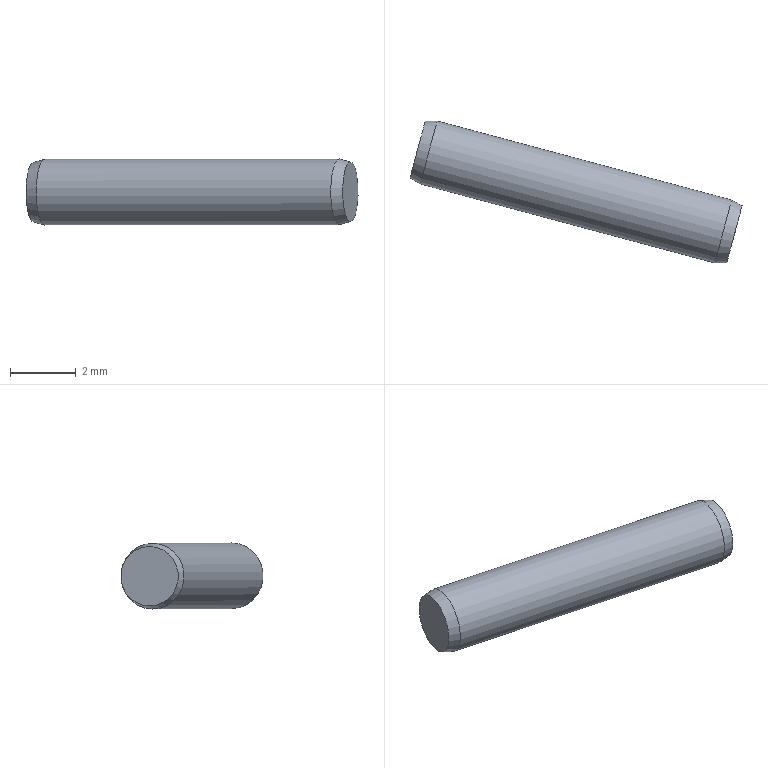Component | NX | GB-T119_1-2000_2X10 | 1 solid | 5 faces | box 10.13 x 4.34 x 2.01 mm | volume 31 mm3 | plane 2 | cone 2 | cylinder 1 | commonest cylinder face diameters 2 x1
STEP:
#1=CARTESIAN_POINT('',(0.,0.,0.));
#2=DIRECTION('',(0.,0.,1.));
#3=DIRECTION('',(1.,0.,0.));
#4=AXIS2_PLACEMENT_3D('',#1,#2,#3);
#5=CARTESIAN_POINT('',(19.96,-124.109,157.371));
#6=VERTEX_POINT('',#5);
#7=CARTESIAN_POINT('',(19.961,-124.109,156.465));
#8=DIRECTION('',(-0.9659,0.2589,-0.001382));
#9=DIRECTION('',(-0.001431,0.,1.));
#10=AXIS2_PLACEMENT_3D('',#7,#8,#9);
#11=CIRCLE('',#10,0.9062);
#12=CARTESIAN_POINT('',(19.961,-124.109,156.465));
#13=DIRECTION('',(-0.9659,0.2589,-0.001382));
#14=DIRECTION('',(-0.001431,-0.,1.));
#15=AXIS2_PLACEMENT_3D('',#12,#13,#14);
#16=PLANE('',#15);
#17=CARTESIAN_POINT('',(0.,0.));
#18=DIRECTION('',(1.,0.));
#19=AXIS2_PLACEMENT_2D('',#17,#18);
#20=CIRCLE('',#19,0.9062);
#21=(GEOMETRIC_REPRESENTATION_CONTEXT(2)PARAMETRIC_REPRESENTATION_CONTEXT()REPRESENTATION_CONTEXT('',''));
#22=DEFINITIONAL_REPRESENTATION('',(#20),#21);
#23=PCURVE('',#16,#22);
#24=CARTESIAN_POINT('',(19.961,-124.109,156.465));
#25=DIRECTION('',(0.9659,-0.2589,0.001382));
#26=DIRECTION('',(0.001431,0.,-1.));
#27=AXIS2_PLACEMENT_3D('',#24,#25,#26);
#28=CONICAL_SURFACE('',#27,0.9062,0.2618);
#29=CARTESIAN_POINT('',(9.425,-0.));
#30=DIRECTION('',(-1.,0.));
#31=VECTOR('',#30,1.);
#32=LINE('',#29,#31);
#33=(GEOMETRIC_REPRESENTATION_CONTEXT(2)PARAMETRIC_REPRESENTATION_CONTEXT()REPRESENTATION_CONTEXT('',''));
#34=DEFINITIONAL_REPRESENTATION('',(#32),#33);
#35=PCURVE('',#28,#34);
#36=SURFACE_CURVE('',#11,(#23,#35),.PCURVE_S1.);
#37=EDGE_CURVE('',#6,#6,#36,.T.);
#38=ORIENTED_EDGE('',*,*,#37,.T.);
#39=EDGE_LOOP('',(#38));
#40=FACE_BOUND('',#39,.T.);
#41=ADVANCED_FACE('',(#40),#16,.T.);
#42=CARTESIAN_POINT('',(20.298,-124.199,157.465));
#43=VERTEX_POINT('',#42);
#44=CARTESIAN_POINT('',(20.299,-124.199,156.465));
#45=DIRECTION('',(-0.9659,0.2589,-0.001382));
#46=DIRECTION('',(-0.001431,-0.,1.));
#47=AXIS2_PLACEMENT_3D('',#44,#45,#46);
#48=CIRCLE('',#47,1.);
#49=CARTESIAN_POINT('',(9.425,0.35));
#50=DIRECTION('',(-1.,0.));
#51=VECTOR('',#50,1.);
#52=LINE('',#49,#51);
#53=(GEOMETRIC_REPRESENTATION_CONTEXT(2)PARAMETRIC_REPRESENTATION_CONTEXT()REPRESENTATION_CONTEXT('',''));
#54=DEFINITIONAL_REPRESENTATION('',(#52),#53);
#55=PCURVE('',#28,#54);
#56=CARTESIAN_POINT('',(29.62,-126.698,156.479));
#57=DIRECTION('',(-0.9659,0.2589,-0.001382));
#58=DIRECTION('',(-0.001431,-0.,1.));
#59=AXIS2_PLACEMENT_3D('',#56,#57,#58);
#60=CYLINDRICAL_SURFACE('',#59,1.);
#61=CARTESIAN_POINT('',(0.,9.65));
#62=DIRECTION('',(1.,0.));
#63=VECTOR('',#62,1.);
#64=LINE('',#61,#63);
#65=(GEOMETRIC_REPRESENTATION_CONTEXT(2)PARAMETRIC_REPRESENTATION_CONTEXT()REPRESENTATION_CONTEXT('',''));
#66=DEFINITIONAL_REPRESENTATION('',(#64),#65);
#67=PCURVE('',#60,#66);
#68=SURFACE_CURVE('',#48,(#55,#67),.PCURVE_S1.);
#69=EDGE_CURVE('',#43,#43,#68,.T.);
#70=ORIENTED_EDGE('',*,*,#69,.T.);
#71=CARTESIAN_POINT('',(19.96,-124.109,157.371));
#72=CARTESIAN_POINT('',(20.298,-124.199,157.465));
#73=B_SPLINE_CURVE_WITH_KNOTS('',1,(#71,#72),.UNSPECIFIED.,.F.,.F.,(2,2),(-0.,0.3623),.PIECEWISE_BEZIER_KNOTS.);
#74=CARTESIAN_POINT('',(3.142,0.));
#75=DIRECTION('',(0.,1.));
#76=VECTOR('',#75,1.);
#77=LINE('',#74,#76);
#78=(GEOMETRIC_REPRESENTATION_CONTEXT(2)PARAMETRIC_REPRESENTATION_CONTEXT()REPRESENTATION_CONTEXT('',''));
#79=DEFINITIONAL_REPRESENTATION('',(#77),#78);
#80=PCURVE('',#28,#79);
#81=CARTESIAN_POINT('',(9.425,0.));
#82=DIRECTION('',(0.,1.));
#83=VECTOR('',#82,1.);
#84=LINE('',#81,#83);
#85=(GEOMETRIC_REPRESENTATION_CONTEXT(2)PARAMETRIC_REPRESENTATION_CONTEXT()REPRESENTATION_CONTEXT('',''));
#86=DEFINITIONAL_REPRESENTATION('',(#84),#85);
#87=PCURVE('',#28,#86);
#88=SEAM_CURVE('',#73,(#80,#87),.PCURVE_S1.);
#89=EDGE_CURVE('',#6,#43,#88,.T.);
#90=ORIENTED_EDGE('',*,*,#89,.F.);
#91=ORIENTED_EDGE('',*,*,#37,.F.);
#92=ORIENTED_EDGE('',*,*,#89,.T.);
#93=EDGE_LOOP('',(#70,#90,#91,#92));
#94=FACE_BOUND('',#93,.T.);
#95=ADVANCED_FACE('',(#94),#28,.T.);
#96=CARTESIAN_POINT('',(29.281,-126.607,157.478));
#97=VERTEX_POINT('',#96);
#98=CARTESIAN_POINT('',(29.282,-126.607,156.478));
#99=DIRECTION('',(-0.9659,0.2589,-0.001382));
#100=DIRECTION('',(-0.001431,-0.,1.));
#101=AXIS2_PLACEMENT_3D('',#98,#99,#100);
#102=CIRCLE('',#101,1.);
#103=CARTESIAN_POINT('',(0.,0.35));
#104=DIRECTION('',(1.,0.));
#105=VECTOR('',#104,1.);
#106=LINE('',#103,#105);
#107=(GEOMETRIC_REPRESENTATION_CONTEXT(2)PARAMETRIC_REPRESENTATION_CONTEXT()REPRESENTATION_CONTEXT('',''));
#108=DEFINITIONAL_REPRESENTATION('',(#106),#107);
#109=PCURVE('',#60,#108);
#110=CARTESIAN_POINT('',(29.282,-126.607,156.478));
#111=DIRECTION('',(-0.9659,0.2589,-0.001382));
#112=DIRECTION('',(-0.001431,-0.,1.));
#113=AXIS2_PLACEMENT_3D('',#110,#111,#112);
#114=CONICAL_SURFACE('',#113,1.,0.2618);
#115=CARTESIAN_POINT('',(0.,-0.));
#116=DIRECTION('',(1.,0.));
#117=VECTOR('',#116,1.);
#118=LINE('',#115,#117);
#119=(GEOMETRIC_REPRESENTATION_CONTEXT(2)PARAMETRIC_REPRESENTATION_CONTEXT()REPRESENTATION_CONTEXT('',''));
#120=DEFINITIONAL_REPRESENTATION('',(#118),#119);
#121=PCURVE('',#114,#120);
#122=SURFACE_CURVE('',#102,(#109,#121),.PCURVE_S1.);
#123=EDGE_CURVE('',#97,#97,#122,.T.);
#124=ORIENTED_EDGE('',*,*,#123,.T.);
#125=CARTESIAN_POINT('',(29.281,-126.607,157.478));
#126=CARTESIAN_POINT('',(20.298,-124.199,157.465));
#127=B_SPLINE_CURVE_WITH_KNOTS('',1,(#125,#126),.UNSPECIFIED.,.F.,.F.,(2,2),(0.35,9.65),.PIECEWISE_BEZIER_KNOTS.);
#128=CARTESIAN_POINT('',(6.283,0.));
#129=DIRECTION('',(0.,1.));
#130=VECTOR('',#129,1.);
#131=LINE('',#128,#130);
#132=(GEOMETRIC_REPRESENTATION_CONTEXT(2)PARAMETRIC_REPRESENTATION_CONTEXT()REPRESENTATION_CONTEXT('',''));
#133=DEFINITIONAL_REPRESENTATION('',(#131),#132);
#134=PCURVE('',#60,#133);
#135=CARTESIAN_POINT('',(0.,0.));
#136=DIRECTION('',(0.,1.));
#137=VECTOR('',#136,1.);
#138=LINE('',#135,#137);
#139=(GEOMETRIC_REPRESENTATION_CONTEXT(2)PARAMETRIC_REPRESENTATION_CONTEXT()REPRESENTATION_CONTEXT('',''));
#140=DEFINITIONAL_REPRESENTATION('',(#138),#139);
#141=PCURVE('',#60,#140);
#142=SEAM_CURVE('',#127,(#134,#141),.PCURVE_S1.);
#143=EDGE_CURVE('',#97,#43,#142,.T.);
#144=ORIENTED_EDGE('',*,*,#143,.T.);
#145=ORIENTED_EDGE('',*,*,#69,.F.);
#146=ORIENTED_EDGE('',*,*,#143,.F.);
#147=EDGE_LOOP('',(#124,#144,#145,#146));
#148=FACE_BOUND('',#147,.T.);
#149=ADVANCED_FACE('',(#148),#60,.T.);
#150=CARTESIAN_POINT('',(29.619,-126.698,157.385));
#151=VERTEX_POINT('',#150);
#152=CARTESIAN_POINT('',(29.62,-126.698,156.479));
#153=DIRECTION('',(-0.9659,0.2589,-0.001382));
#154=DIRECTION('',(-0.001431,0.,1.));
#155=AXIS2_PLACEMENT_3D('',#152,#153,#154);
#156=CIRCLE('',#155,0.9062);
#157=CARTESIAN_POINT('',(0.,-0.35));
#158=DIRECTION('',(1.,0.));
#159=VECTOR('',#158,1.);
#160=LINE('',#157,#159);
#161=(GEOMETRIC_REPRESENTATION_CONTEXT(2)PARAMETRIC_REPRESENTATION_CONTEXT()REPRESENTATION_CONTEXT('',''));
#162=DEFINITIONAL_REPRESENTATION('',(#160),#161);
#163=PCURVE('',#114,#162);
#164=CARTESIAN_POINT('',(29.621,-126.698,155.572));
#165=DIRECTION('',(0.9659,-0.2589,0.001382));
#166=DIRECTION('',(0.001431,0.,-1.));
#167=AXIS2_PLACEMENT_3D('',#164,#165,#166);
#168=PLANE('',#167);
#169=CARTESIAN_POINT('',(-1.812,0.));
#170=CARTESIAN_POINT('',(-1.812,1.57));
#171=CARTESIAN_POINT('',(-0.4531,0.7848));
#172=CARTESIAN_POINT('',(0.9062,-0.));
#173=CARTESIAN_POINT('',(-0.4531,-0.7848));
#174=CARTESIAN_POINT('',(-1.812,-1.57));
#175=CARTESIAN_POINT('',(-1.812,0.));
#176=(BOUNDED_CURVE()B_SPLINE_CURVE(2,(#169,#170,#171,#172,#173,#174,#175),.UNSPECIFIED.,.T.,.F.)B_SPLINE_CURVE_WITH_KNOTS((1,2,2,2,2,1),(-2.094,0.,2.094,4.189,6.283,8.378),.UNSPECIFIED.)CURVE()GEOMETRIC_REPRESENTATION_ITEM()RATIONAL_B_SPLINE_CURVE((1.,0.5,1.,0.5,1.,0.5,1.))REPRESENTATION_ITEM(''));
#177=(GEOMETRIC_REPRESENTATION_CONTEXT(2)PARAMETRIC_REPRESENTATION_CONTEXT()REPRESENTATION_CONTEXT('',''));
#178=DEFINITIONAL_REPRESENTATION('',(#176),#177);
#179=PCURVE('',#168,#178);
#180=SURFACE_CURVE('',#156,(#163,#179),.PCURVE_S1.);
#181=EDGE_CURVE('',#151,#151,#180,.T.);
#182=ORIENTED_EDGE('',*,*,#181,.T.);
#183=CARTESIAN_POINT('',(29.619,-126.698,157.385));
#184=CARTESIAN_POINT('',(29.281,-126.607,157.478));
#185=B_SPLINE_CURVE_WITH_KNOTS('',1,(#183,#184),.UNSPECIFIED.,.F.,.F.,(2,2),(-0.3623,-0.),.PIECEWISE_BEZIER_KNOTS.);
#186=CARTESIAN_POINT('',(6.283,0.));
#187=DIRECTION('',(0.,1.));
#188=VECTOR('',#187,1.);
#189=LINE('',#186,#188);
#190=(GEOMETRIC_REPRESENTATION_CONTEXT(2)PARAMETRIC_REPRESENTATION_CONTEXT()REPRESENTATION_CONTEXT('',''));
#191=DEFINITIONAL_REPRESENTATION('',(#189),#190);
#192=PCURVE('',#114,#191);
#193=CARTESIAN_POINT('',(0.,0.));
#194=DIRECTION('',(0.,1.));
#195=VECTOR('',#194,1.);
#196=LINE('',#193,#195);
#197=(GEOMETRIC_REPRESENTATION_CONTEXT(2)PARAMETRIC_REPRESENTATION_CONTEXT()REPRESENTATION_CONTEXT('',''));
#198=DEFINITIONAL_REPRESENTATION('',(#196),#197);
#199=PCURVE('',#114,#198);
#200=SEAM_CURVE('',#185,(#192,#199),.PCURVE_S1.);
#201=EDGE_CURVE('',#151,#97,#200,.T.);
#202=ORIENTED_EDGE('',*,*,#201,.T.);
#203=ORIENTED_EDGE('',*,*,#123,.F.);
#204=ORIENTED_EDGE('',*,*,#201,.F.);
#205=EDGE_LOOP('',(#182,#202,#203,#204));
#206=FACE_BOUND('',#205,.T.);
#207=ADVANCED_FACE('',(#206),#114,.T.);
#208=ORIENTED_EDGE('',*,*,#181,.F.);
#209=EDGE_LOOP('',(#208));
#210=FACE_BOUND('',#209,.T.);
#211=ADVANCED_FACE('',(#210),#168,.T.);
#212=CLOSED_SHELL('',(#41,#95,#149,#207,#211));
#213=MANIFOLD_SOLID_BREP('',#212);
#214=(LENGTH_UNIT()NAMED_UNIT(*)SI_UNIT(.MILLI.,.METRE.));
#215=UNCERTAINTY_MEASURE_WITH_UNIT(LENGTH_MEASURE(0.00001),#214,'','');
#216=(NAMED_UNIT(*)PLANE_ANGLE_UNIT()SI_UNIT($,.RADIAN.));
#217=(NAMED_UNIT(*)SI_UNIT($,.STERADIAN.)SOLID_ANGLE_UNIT());
#218=(GEOMETRIC_REPRESENTATION_CONTEXT(3)GLOBAL_UNCERTAINTY_ASSIGNED_CONTEXT((#215))GLOBAL_UNIT_ASSIGNED_CONTEXT((#214,#216,#217))REPRESENTATION_CONTEXT('',''));
#219=ADVANCED_BREP_SHAPE_REPRESENTATION('',(#4,#213),#218);